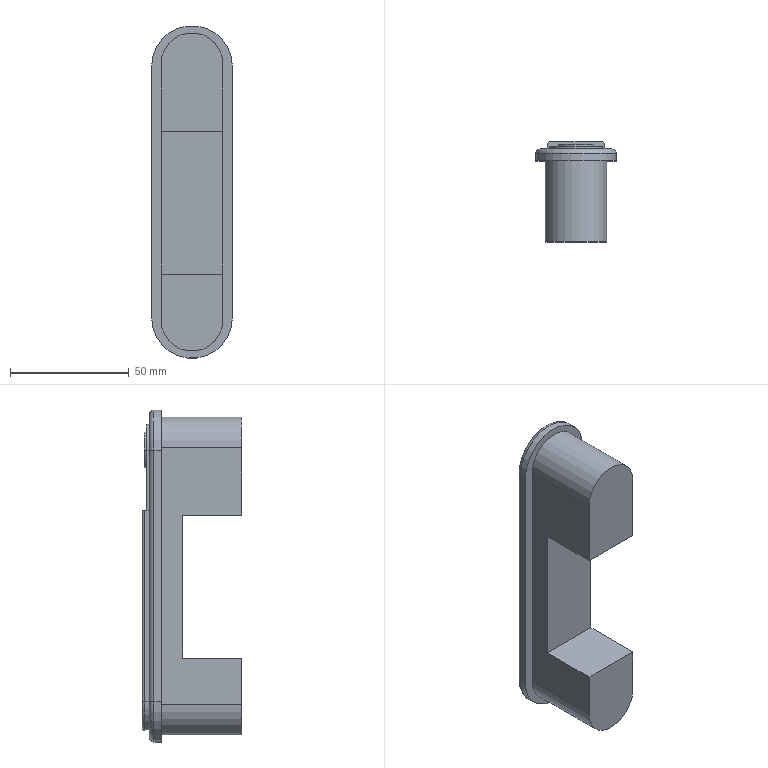Component | SolidWorks | OuterDoorAssembly1-1_MMS480-2A-1Lock-1 | 1 solid | 39 faces | box 34 x 42.01 x 140 mm | volume 104134 mm3 | plane 24 | cylinder 12 | torus 3 | commonest cylinder face diameters 15 x2 34 x2 4 x2 2 x2 26 x2 24 x1 22 x1
STEP:
#1=CARTESIAN_POINT('',(-2.264,7.503,34.753));
#2=VERTEX_POINT('',#1);
#3=CARTESIAN_POINT('',(-2.854,7.503,34.753));
#4=VERTEX_POINT('',#3);
#5=CARTESIAN_POINT('',(-2.559,7.503,34.753));
#6=DIRECTION('',(0.0003491,1.,-0.));
#7=DIRECTION('',(1.,-0.0003491,0.));
#8=AXIS2_PLACEMENT_3D('',#5,#6,#7);
#9=CIRCLE('',#8,0.2953);
#10=EDGE_CURVE('',#2,#4,#9,.T.);
#11=ORIENTED_EDGE('',*,*,#10,.F.);
#12=CARTESIAN_POINT('',(-2.264,7.463,34.753));
#13=VERTEX_POINT('',#12);
#14=CARTESIAN_POINT('',(-2.264,7.503,34.753));
#15=DIRECTION('',(-0.0003491,-1.,0.));
#16=VECTOR('',#15,39.37);
#17=LINE('',#14,#16);
#18=EDGE_CURVE('',#2,#13,#17,.T.);
#19=ORIENTED_EDGE('',*,*,#18,.T.);
#20=CARTESIAN_POINT('',(-2.854,7.463,34.753));
#21=VERTEX_POINT('',#20);
#22=CARTESIAN_POINT('',(-2.559,7.463,34.753));
#23=DIRECTION('',(0.0003491,1.,-0.));
#24=DIRECTION('',(1.,-0.0003491,0.));
#25=AXIS2_PLACEMENT_3D('',#22,#23,#24);
#26=CIRCLE('',#25,0.2953);
#27=EDGE_CURVE('',#13,#21,#26,.T.);
#28=ORIENTED_EDGE('',*,*,#27,.T.);
#29=CARTESIAN_POINT('',(-2.854,7.503,34.753));
#30=DIRECTION('',(-0.0003491,-1.,0.));
#31=VECTOR('',#30,39.37);
#32=LINE('',#29,#31);
#33=EDGE_CURVE('',#4,#21,#32,.T.);
#34=ORIENTED_EDGE('',*,*,#33,.F.);
#35=EDGE_LOOP('',(#11,#19,#28,#34));
#36=FACE_OUTER_BOUND('',#35,.T.);
#37=CARTESIAN_POINT('',(-2.559,7.503,34.753));
#38=DIRECTION('',(-0.0003491,-1.,0.));
#39=DIRECTION('',(-1.,0.0003491,0.));
#40=AXIS2_PLACEMENT_3D('',#37,#38,#39);
#41=CYLINDRICAL_SURFACE('',#40,0.2953);
#42=ADVANCED_FACE('',(#36),#41,.T.);
#43=CARTESIAN_POINT('',(-2.048,5.888,30.54));
#44=VERTEX_POINT('',#43);
#45=CARTESIAN_POINT('',(-2.048,5.888,31.307));
#46=VERTEX_POINT('',#45);
#47=CARTESIAN_POINT('',(-2.048,5.888,30.54));
#48=DIRECTION('',(-0.,0.,1.));
#49=VECTOR('',#48,39.37);
#50=LINE('',#47,#49);
#51=EDGE_CURVE('',#44,#46,#50,.T.);
#52=ORIENTED_EDGE('',*,*,#51,.T.);
#53=CARTESIAN_POINT('',(-3.071,5.889,31.307));
#54=VERTEX_POINT('',#53);
#55=CARTESIAN_POINT('',(-2.56,5.888,31.307));
#56=DIRECTION('',(1.,-0.0003491,0.));
#57=VECTOR('',#56,39.37);
#58=LINE('',#55,#57);
#59=EDGE_CURVE('',#54,#46,#58,.T.);
#60=ORIENTED_EDGE('',*,*,#59,.F.);
#61=CARTESIAN_POINT('',(-3.071,5.889,30.54));
#62=VERTEX_POINT('',#61);
#63=CARTESIAN_POINT('',(-3.071,5.889,30.54));
#64=DIRECTION('',(0.,-0.,-1.));
#65=VECTOR('',#64,39.37);
#66=LINE('',#63,#65);
#67=EDGE_CURVE('',#54,#62,#66,.T.);
#68=ORIENTED_EDGE('',*,*,#67,.T.);
#69=CARTESIAN_POINT('',(-2.56,5.888,30.54));
#70=DIRECTION('',(-0.0003491,-1.,0.));
#71=DIRECTION('',(-1.,0.0003491,0.));
#72=AXIS2_PLACEMENT_3D('',#69,#70,#71);
#73=CIRCLE('',#72,0.5118);
#74=EDGE_CURVE('',#62,#44,#73,.T.);
#75=ORIENTED_EDGE('',*,*,#74,.T.);
#76=EDGE_LOOP('',(#52,#60,#68,#75));
#77=FACE_OUTER_BOUND('',#76,.T.);
#78=CARTESIAN_POINT('',(-2.56,5.888,30.54));
#79=DIRECTION('',(-0.0003491,-1.,0.));
#80=DIRECTION('',(-1.,0.0003491,-0.));
#81=AXIS2_PLACEMENT_3D('',#78,#79,#80);
#82=PLANE('',#81);
#83=ADVANCED_FACE('',(#77),#82,.T.);
#84=CARTESIAN_POINT('',(-1.89,7.227,30.58));
#85=VERTEX_POINT('',#84);
#86=CARTESIAN_POINT('',(-3.228,7.227,30.58));
#87=VERTEX_POINT('',#86);
#88=CARTESIAN_POINT('',(-2.559,7.227,30.58));
#89=DIRECTION('',(0.0003491,1.,-0.));
#90=DIRECTION('',(1.,-0.0003491,0.));
#91=AXIS2_PLACEMENT_3D('',#88,#89,#90);
#92=CIRCLE('',#91,0.6693);
#93=EDGE_CURVE('',#85,#87,#92,.T.);
#94=ORIENTED_EDGE('',*,*,#93,.F.);
#95=CARTESIAN_POINT('',(-1.89,7.227,34.753));
#96=VERTEX_POINT('',#95);
#97=CARTESIAN_POINT('',(-1.89,7.227,30.58));
#98=DIRECTION('',(0.,-0.,-1.));
#99=VECTOR('',#98,39.37);
#100=LINE('',#97,#99);
#101=EDGE_CURVE('',#96,#85,#100,.T.);
#102=ORIENTED_EDGE('',*,*,#101,.F.);
#103=CARTESIAN_POINT('',(-3.228,7.227,34.753));
#104=VERTEX_POINT('',#103);
#105=CARTESIAN_POINT('',(-2.559,7.227,34.753));
#106=DIRECTION('',(0.0003491,1.,-0.));
#107=DIRECTION('',(1.,-0.0003491,0.));
#108=AXIS2_PLACEMENT_3D('',#105,#106,#107);
#109=CIRCLE('',#108,0.6693);
#110=EDGE_CURVE('',#104,#96,#109,.T.);
#111=ORIENTED_EDGE('',*,*,#110,.F.);
#112=CARTESIAN_POINT('',(-3.228,7.227,30.58));
#113=DIRECTION('',(-0.,0.,1.));
#114=VECTOR('',#113,39.37);
#115=LINE('',#112,#114);
#116=EDGE_CURVE('',#87,#104,#115,.T.);
#117=ORIENTED_EDGE('',*,*,#116,.F.);
#118=EDGE_LOOP('',(#94,#102,#111,#117));
#119=FACE_OUTER_BOUND('',#118,.T.);
#120=CARTESIAN_POINT('',(-3.071,7.227,30.54));
#121=VERTEX_POINT('',#120);
#122=CARTESIAN_POINT('',(-2.047,7.227,30.54));
#123=VERTEX_POINT('',#122);
#124=CARTESIAN_POINT('',(-2.559,7.227,30.54));
#125=DIRECTION('',(-0.0003491,-1.,0.));
#126=DIRECTION('',(-1.,0.0003491,0.));
#127=AXIS2_PLACEMENT_3D('',#124,#125,#126);
#128=CIRCLE('',#127,0.5118);
#129=EDGE_CURVE('',#121,#123,#128,.T.);
#130=ORIENTED_EDGE('',*,*,#129,.F.);
#131=CARTESIAN_POINT('',(-3.071,7.227,34.792));
#132=VERTEX_POINT('',#131);
#133=CARTESIAN_POINT('',(-3.071,7.227,30.54));
#134=DIRECTION('',(0.,-0.,-1.));
#135=VECTOR('',#134,39.37);
#136=LINE('',#133,#135);
#137=EDGE_CURVE('',#132,#121,#136,.T.);
#138=ORIENTED_EDGE('',*,*,#137,.F.);
#139=CARTESIAN_POINT('',(-2.047,7.227,34.792));
#140=VERTEX_POINT('',#139);
#141=CARTESIAN_POINT('',(-2.559,7.227,34.792));
#142=DIRECTION('',(-0.0003491,-1.,0.));
#143=DIRECTION('',(-1.,0.0003491,0.));
#144=AXIS2_PLACEMENT_3D('',#141,#142,#143);
#145=CIRCLE('',#144,0.5118);
#146=EDGE_CURVE('',#140,#132,#145,.T.);
#147=ORIENTED_EDGE('',*,*,#146,.F.);
#148=CARTESIAN_POINT('',(-2.047,7.227,30.54));
#149=DIRECTION('',(-0.,0.,1.));
#150=VECTOR('',#149,39.37);
#151=LINE('',#148,#150);
#152=EDGE_CURVE('',#123,#140,#151,.T.);
#153=ORIENTED_EDGE('',*,*,#152,.F.);
#154=EDGE_LOOP('',(#130,#138,#147,#153));
#155=FACE_BOUND('',#154,.T.);
#156=CARTESIAN_POINT('',(-2.559,7.227,30.58));
#157=DIRECTION('',(0.0003491,1.,-0.));
#158=DIRECTION('',(1.,-0.0003491,0.));
#159=AXIS2_PLACEMENT_3D('',#156,#157,#158);
#160=PLANE('',#159);
#161=ADVANCED_FACE('',(#119,#155),#160,.F.);
#162=CARTESIAN_POINT('',(-2.992,7.463,33.745));
#163=VERTEX_POINT('',#162);
#164=CARTESIAN_POINT('',(-2.126,7.463,33.745));
#165=VERTEX_POINT('',#164);
#166=CARTESIAN_POINT('',(-3.031,7.463,33.745));
#167=DIRECTION('',(1.,-0.0003491,0.));
#168=VECTOR('',#167,39.37);
#169=LINE('',#166,#168);
#170=EDGE_CURVE('',#163,#165,#169,.T.);
#171=ORIENTED_EDGE('',*,*,#170,.F.);
#172=CARTESIAN_POINT('',(-2.992,7.463,34.753));
#173=VERTEX_POINT('',#172);
#174=CARTESIAN_POINT('',(-2.992,7.463,34.753));
#175=DIRECTION('',(-0.,0.,1.));
#176=VECTOR('',#175,39.37);
#177=LINE('',#174,#176);
#178=EDGE_CURVE('',#163,#173,#177,.T.);
#179=ORIENTED_EDGE('',*,*,#178,.T.);
#180=CARTESIAN_POINT('',(-2.126,7.463,34.753));
#181=VERTEX_POINT('',#180);
#182=CARTESIAN_POINT('',(-2.559,7.463,34.753));
#183=DIRECTION('',(0.0003491,1.,-0.));
#184=DIRECTION('',(1.,-0.0003491,0.));
#185=AXIS2_PLACEMENT_3D('',#182,#183,#184);
#186=CIRCLE('',#185,0.4331);
#187=EDGE_CURVE('',#173,#181,#186,.T.);
#188=ORIENTED_EDGE('',*,*,#187,.T.);
#189=CARTESIAN_POINT('',(-2.126,7.463,34.753));
#190=DIRECTION('',(0.,-0.,-1.));
#191=VECTOR('',#190,39.37);
#192=LINE('',#189,#191);
#193=EDGE_CURVE('',#181,#165,#192,.T.);
#194=ORIENTED_EDGE('',*,*,#193,.T.);
#195=EDGE_LOOP('',(#171,#179,#188,#194));
#196=FACE_OUTER_BOUND('',#195,.T.);
#197=CARTESIAN_POINT('',(-2.559,7.463,34.753));
#198=DIRECTION('',(0.0003491,1.,-0.));
#199=DIRECTION('',(1.,-0.0003491,0.));
#200=AXIS2_PLACEMENT_3D('',#197,#198,#199);
#201=CIRCLE('',#200,0.2953);
#202=EDGE_CURVE('',#21,#13,#201,.T.);
#203=ORIENTED_EDGE('',*,*,#202,.F.);
#204=ORIENTED_EDGE('',*,*,#27,.F.);
#205=EDGE_LOOP('',(#203,#204));
#206=FACE_BOUND('',#205,.T.);
#207=CARTESIAN_POINT('',(-2.559,7.463,34.753));
#208=DIRECTION('',(0.0003491,1.,-0.));
#209=DIRECTION('',(1.,-0.0003491,0.));
#210=AXIS2_PLACEMENT_3D('',#207,#208,#209);
#211=PLANE('',#210);
#212=ADVANCED_FACE('',(#196,#206),#211,.T.);
#213=CARTESIAN_POINT('',(-3.15,7.424,34.753));
#214=VERTEX_POINT('',#213);
#215=CARTESIAN_POINT('',(-1.968,7.424,34.753));
#216=VERTEX_POINT('',#215);
#217=CARTESIAN_POINT('',(-2.559,7.424,34.753));
#218=DIRECTION('',(0.0003491,1.,-0.));
#219=DIRECTION('',(1.,-0.0003491,0.));
#220=AXIS2_PLACEMENT_3D('',#217,#218,#219);
#221=CIRCLE('',#220,0.5906);
#222=EDGE_CURVE('',#214,#216,#221,.T.);
#223=ORIENTED_EDGE('',*,*,#222,.T.);
#224=CARTESIAN_POINT('',(-1.968,7.424,30.58));
#225=VERTEX_POINT('',#224);
#226=CARTESIAN_POINT('',(-1.968,7.424,30.58));
#227=DIRECTION('',(0.,-0.,-1.));
#228=VECTOR('',#227,39.37);
#229=LINE('',#226,#228);
#230=EDGE_CURVE('',#216,#225,#229,.T.);
#231=ORIENTED_EDGE('',*,*,#230,.T.);
#232=CARTESIAN_POINT('',(-3.15,7.424,30.58));
#233=VERTEX_POINT('',#232);
#234=CARTESIAN_POINT('',(-2.559,7.424,30.58));
#235=DIRECTION('',(0.0003491,1.,-0.));
#236=DIRECTION('',(1.,-0.0003491,0.));
#237=AXIS2_PLACEMENT_3D('',#234,#235,#236);
#238=CIRCLE('',#237,0.5906);
#239=EDGE_CURVE('',#225,#233,#238,.T.);
#240=ORIENTED_EDGE('',*,*,#239,.T.);
#241=CARTESIAN_POINT('',(-3.15,7.424,34.753));
#242=DIRECTION('',(-0.,0.,1.));
#243=VECTOR('',#242,39.37);
#244=LINE('',#241,#243);
#245=EDGE_CURVE('',#233,#214,#244,.T.);
#246=ORIENTED_EDGE('',*,*,#245,.T.);
#247=EDGE_LOOP('',(#223,#231,#240,#246));
#248=FACE_OUTER_BOUND('',#247,.T.);
#249=CARTESIAN_POINT('',(-2.126,7.424,33.745));
#250=VERTEX_POINT('',#249);
#251=CARTESIAN_POINT('',(-2.087,7.424,33.745));
#252=VERTEX_POINT('',#251);
#253=CARTESIAN_POINT('',(-3.031,7.424,33.745));
#254=DIRECTION('',(1.,-0.0003491,0.));
#255=VECTOR('',#254,39.37);
#256=LINE('',#253,#255);
#257=EDGE_CURVE('',#250,#252,#256,.T.);
#258=ORIENTED_EDGE('',*,*,#257,.F.);
#259=CARTESIAN_POINT('',(-2.126,7.424,34.753));
#260=VERTEX_POINT('',#259);
#261=CARTESIAN_POINT('',(-2.126,7.424,34.753));
#262=DIRECTION('',(0.,-0.,-1.));
#263=VECTOR('',#262,39.37);
#264=LINE('',#261,#263);
#265=EDGE_CURVE('',#260,#250,#264,.T.);
#266=ORIENTED_EDGE('',*,*,#265,.F.);
#267=CARTESIAN_POINT('',(-2.992,7.424,34.753));
#268=VERTEX_POINT('',#267);
#269=CARTESIAN_POINT('',(-2.559,7.424,34.753));
#270=DIRECTION('',(0.0003491,1.,-0.));
#271=DIRECTION('',(1.,-0.0003491,0.));
#272=AXIS2_PLACEMENT_3D('',#269,#270,#271);
#273=CIRCLE('',#272,0.4331);
#274=EDGE_CURVE('',#268,#260,#273,.T.);
#275=ORIENTED_EDGE('',*,*,#274,.F.);
#276=CARTESIAN_POINT('',(-2.992,7.424,33.745));
#277=VERTEX_POINT('',#276);
#278=CARTESIAN_POINT('',(-2.992,7.424,34.753));
#279=DIRECTION('',(-0.,0.,1.));
#280=VECTOR('',#279,39.37);
#281=LINE('',#278,#280);
#282=EDGE_CURVE('',#277,#268,#281,.T.);
#283=ORIENTED_EDGE('',*,*,#282,.F.);
#284=CARTESIAN_POINT('',(-3.031,7.424,33.745));
#285=VERTEX_POINT('',#284);
#286=CARTESIAN_POINT('',(-3.031,7.424,33.745));
#287=DIRECTION('',(1.,-0.0003491,0.));
#288=VECTOR('',#287,39.37);
#289=LINE('',#286,#288);
#290=EDGE_CURVE('',#285,#277,#289,.T.);
#291=ORIENTED_EDGE('',*,*,#290,.F.);
#292=CARTESIAN_POINT('',(-3.031,7.424,30.58));
#293=VERTEX_POINT('',#292);
#294=CARTESIAN_POINT('',(-3.031,7.424,30.58));
#295=DIRECTION('',(-0.,0.,1.));
#296=VECTOR('',#295,39.37);
#297=LINE('',#294,#296);
#298=EDGE_CURVE('',#293,#285,#297,.T.);
#299=ORIENTED_EDGE('',*,*,#298,.F.);
#300=CARTESIAN_POINT('',(-2.087,7.424,30.58));
#301=VERTEX_POINT('',#300);
#302=CARTESIAN_POINT('',(-2.559,7.424,30.58));
#303=DIRECTION('',(0.0003491,1.,-0.));
#304=DIRECTION('',(1.,-0.0003491,0.));
#305=AXIS2_PLACEMENT_3D('',#302,#303,#304);
#306=CIRCLE('',#305,0.4724);
#307=EDGE_CURVE('',#301,#293,#306,.T.);
#308=ORIENTED_EDGE('',*,*,#307,.F.);
#309=CARTESIAN_POINT('',(-2.087,7.424,30.58));
#310=DIRECTION('',(0.,-0.,-1.));
#311=VECTOR('',#310,39.37);
#312=LINE('',#309,#311);
#313=EDGE_CURVE('',#252,#301,#312,.T.);
#314=ORIENTED_EDGE('',*,*,#313,.F.);
#315=EDGE_LOOP('',(#258,#266,#275,#283,#291,#299,#308,#314));
#316=FACE_BOUND('',#315,.T.);
#317=CARTESIAN_POINT('',(-2.559,7.424,30.58));
#318=DIRECTION('',(0.0003491,1.,-0.));
#319=DIRECTION('',(1.,-0.0003491,0.));
#320=AXIS2_PLACEMENT_3D('',#317,#318,#319);
#321=PLANE('',#320);
#322=ADVANCED_FACE('',(#248,#316),#321,.T.);
#323=CARTESIAN_POINT('',(-2.087,7.502,33.745));
#324=VERTEX_POINT('',#323);
#325=CARTESIAN_POINT('',(-2.087,7.542,33.745));
#326=DIRECTION('',(-0.0003491,-1.,0.));
#327=VECTOR('',#326,39.37);
#328=LINE('',#325,#327);
#329=EDGE_CURVE('',#324,#252,#328,.T.);
#330=ORIENTED_EDGE('',*,*,#329,.F.);
#331=CARTESIAN_POINT('',(-2.126,7.542,33.745));
#332=VERTEX_POINT('',#331);
#333=CARTESIAN_POINT('',(-2.126,7.502,33.745));
#334=DIRECTION('',(-0.,0.,1.));
#335=DIRECTION('',(0.0003491,1.,0.));
#336=AXIS2_PLACEMENT_3D('',#333,#334,#335);
#337=CIRCLE('',#336,0.03937);
#338=EDGE_CURVE('',#324,#332,#337,.T.);
#339=ORIENTED_EDGE('',*,*,#338,.T.);
#340=CARTESIAN_POINT('',(-2.992,7.542,33.745));
#341=VERTEX_POINT('',#340);
#342=CARTESIAN_POINT('',(-3.031,7.542,33.745));
#343=DIRECTION('',(1.,-0.0003491,0.));
#344=VECTOR('',#343,39.37);
#345=LINE('',#342,#344);
#346=EDGE_CURVE('',#341,#332,#345,.T.);
#347=ORIENTED_EDGE('',*,*,#346,.F.);
#348=CARTESIAN_POINT('',(-3.031,7.503,33.745));
#349=VERTEX_POINT('',#348);
#350=CARTESIAN_POINT('',(-2.992,7.503,33.745));
#351=DIRECTION('',(-0.,0.,1.));
#352=DIRECTION('',(0.0003491,1.,0.));
#353=AXIS2_PLACEMENT_3D('',#350,#351,#352);
#354=CIRCLE('',#353,0.03937);
#355=EDGE_CURVE('',#341,#349,#354,.T.);
#356=ORIENTED_EDGE('',*,*,#355,.T.);
#357=CARTESIAN_POINT('',(-3.031,7.542,33.745));
#358=DIRECTION('',(-0.0003491,-1.,0.));
#359=VECTOR('',#358,39.37);
#360=LINE('',#357,#359);
#361=EDGE_CURVE('',#349,#285,#360,.T.);
#362=ORIENTED_EDGE('',*,*,#361,.T.);
#363=ORIENTED_EDGE('',*,*,#290,.T.);
#364=CARTESIAN_POINT('',(-2.992,7.542,33.745));
#365=DIRECTION('',(-0.0003491,-1.,0.));
#366=VECTOR('',#365,39.37);
#367=LINE('',#364,#366);
#368=EDGE_CURVE('',#163,#277,#367,.T.);
#369=ORIENTED_EDGE('',*,*,#368,.F.);
#370=ORIENTED_EDGE('',*,*,#170,.T.);
#371=CARTESIAN_POINT('',(-2.126,7.542,33.745));
#372=DIRECTION('',(0.0003491,1.,-0.));
#373=VECTOR('',#372,39.37);
#374=LINE('',#371,#373);
#375=EDGE_CURVE('',#250,#165,#374,.T.);
#376=ORIENTED_EDGE('',*,*,#375,.F.);
#377=ORIENTED_EDGE('',*,*,#257,.T.);
#378=EDGE_LOOP('',(#330,#339,#347,#356,#362,#363,#369,#370,#376,#377));
#379=FACE_OUTER_BOUND('',#378,.T.);
#380=CARTESIAN_POINT('',(-3.031,7.542,33.745));
#381=DIRECTION('',(0.,-0.,-1.));
#382=DIRECTION('',(0.0003491,1.,-0.));
#383=AXIS2_PLACEMENT_3D('',#380,#381,#382);
#384=PLANE('',#383);
#385=ADVANCED_FACE('',(#379),#384,.F.);
#386=CARTESIAN_POINT('',(-3.228,7.345,30.58));
#387=VERTEX_POINT('',#386);
#388=CARTESIAN_POINT('',(-3.228,7.424,30.58));
#389=DIRECTION('',(-0.0003491,-1.,0.));
#390=VECTOR('',#389,39.37);
#391=LINE('',#388,#390);
#392=EDGE_CURVE('',#387,#87,#391,.T.);
#393=ORIENTED_EDGE('',*,*,#392,.F.);
#394=CARTESIAN_POINT('',(-1.89,7.345,30.58));
#395=VERTEX_POINT('',#394);
#396=CARTESIAN_POINT('',(-2.559,7.345,30.58));
#397=DIRECTION('',(-0.0003491,-1.,0.));
#398=DIRECTION('',(1.,-0.0003491,0.));
#399=AXIS2_PLACEMENT_3D('',#396,#397,#398);
#400=CIRCLE('',#399,0.6693);
#401=EDGE_CURVE('',#387,#395,#400,.T.);
#402=ORIENTED_EDGE('',*,*,#401,.T.);
#403=CARTESIAN_POINT('',(-1.89,7.424,30.58));
#404=DIRECTION('',(-0.0003491,-1.,0.));
#405=VECTOR('',#404,39.37);
#406=LINE('',#403,#405);
#407=EDGE_CURVE('',#395,#85,#406,.T.);
#408=ORIENTED_EDGE('',*,*,#407,.T.);
#409=ORIENTED_EDGE('',*,*,#93,.T.);
#410=EDGE_LOOP('',(#393,#402,#408,#409));
#411=FACE_OUTER_BOUND('',#410,.T.);
#412=CARTESIAN_POINT('',(-2.559,7.424,30.58));
#413=DIRECTION('',(-0.0003491,-1.,0.));
#414=DIRECTION('',(-1.,0.0003491,-0.));
#415=AXIS2_PLACEMENT_3D('',#412,#413,#414);
#416=CYLINDRICAL_SURFACE('',#415,0.6693);
#417=ADVANCED_FACE('',(#411),#416,.T.);
#418=CARTESIAN_POINT('',(-3.228,7.345,34.753));
#419=VERTEX_POINT('',#418);
#420=CARTESIAN_POINT('',(-3.228,7.424,34.753));
#421=DIRECTION('',(-0.0003491,-1.,0.));
#422=VECTOR('',#421,39.37);
#423=LINE('',#420,#422);
#424=EDGE_CURVE('',#419,#104,#423,.T.);
#425=ORIENTED_EDGE('',*,*,#424,.F.);
#426=CARTESIAN_POINT('',(-3.228,7.345,30.58));
#427=DIRECTION('',(0.,-0.,-1.));
#428=VECTOR('',#427,39.37);
#429=LINE('',#426,#428);
#430=EDGE_CURVE('',#419,#387,#429,.T.);
#431=ORIENTED_EDGE('',*,*,#430,.T.);
#432=ORIENTED_EDGE('',*,*,#392,.T.);
#433=ORIENTED_EDGE('',*,*,#116,.T.);
#434=EDGE_LOOP('',(#425,#431,#432,#433));
#435=FACE_OUTER_BOUND('',#434,.T.);
#436=CARTESIAN_POINT('',(-3.228,7.424,30.58));
#437=DIRECTION('',(1.,-0.0003491,0.));
#438=DIRECTION('',(0.,-0.,-1.));
#439=AXIS2_PLACEMENT_3D('',#436,#437,#438);
#440=PLANE('',#439);
#441=ADVANCED_FACE('',(#435),#440,.F.);
#442=CARTESIAN_POINT('',(-1.89,7.345,34.753));
#443=VERTEX_POINT('',#442);
#444=CARTESIAN_POINT('',(-1.89,7.424,34.753));
#445=DIRECTION('',(-0.0003491,-1.,0.));
#446=VECTOR('',#445,39.37);
#447=LINE('',#444,#446);
#448=EDGE_CURVE('',#443,#96,#447,.T.);
#449=ORIENTED_EDGE('',*,*,#448,.F.);
#450=CARTESIAN_POINT('',(-2.559,7.345,34.753));
#451=DIRECTION('',(-0.0003491,-1.,0.));
#452=DIRECTION('',(1.,-0.0003491,0.));
#453=AXIS2_PLACEMENT_3D('',#450,#451,#452);
#454=CIRCLE('',#453,0.6693);
#455=EDGE_CURVE('',#443,#419,#454,.T.);
#456=ORIENTED_EDGE('',*,*,#455,.T.);
#457=ORIENTED_EDGE('',*,*,#424,.T.);
#458=ORIENTED_EDGE('',*,*,#110,.T.);
#459=EDGE_LOOP('',(#449,#456,#457,#458));
#460=FACE_OUTER_BOUND('',#459,.T.);
#461=CARTESIAN_POINT('',(-2.559,7.424,34.753));
#462=DIRECTION('',(-0.0003491,-1.,0.));
#463=DIRECTION('',(-1.,0.0003491,-0.));
#464=AXIS2_PLACEMENT_3D('',#461,#462,#463);
#465=CYLINDRICAL_SURFACE('',#464,0.6693);
#466=ADVANCED_FACE('',(#460),#465,.T.);
#467=ORIENTED_EDGE('',*,*,#407,.F.);
#468=CARTESIAN_POINT('',(-1.89,7.345,34.753));
#469=DIRECTION('',(-0.,0.,1.));
#470=VECTOR('',#469,39.37);
#471=LINE('',#468,#470);
#472=EDGE_CURVE('',#395,#443,#471,.T.);
#473=ORIENTED_EDGE('',*,*,#472,.T.);
#474=ORIENTED_EDGE('',*,*,#448,.T.);
#475=ORIENTED_EDGE('',*,*,#101,.T.);
#476=EDGE_LOOP('',(#467,#473,#474,#475));
#477=FACE_OUTER_BOUND('',#476,.T.);
#478=CARTESIAN_POINT('',(-1.89,7.424,30.58));
#479=DIRECTION('',(-1.,0.0003491,-0.));
#480=DIRECTION('',(-0.,0.,1.));
#481=AXIS2_PLACEMENT_3D('',#478,#479,#480);
#482=PLANE('',#481);
#483=ADVANCED_FACE('',(#477),#482,.F.);
#484=CARTESIAN_POINT('',(-3.031,7.503,30.58));
#485=VERTEX_POINT('',#484);
#486=CARTESIAN_POINT('',(-3.031,7.542,30.58));
#487=DIRECTION('',(-0.0003491,-1.,0.));
#488=VECTOR('',#487,39.37);
#489=LINE('',#486,#488);
#490=EDGE_CURVE('',#485,#293,#489,.T.);
#491=ORIENTED_EDGE('',*,*,#490,.F.);
#492=CARTESIAN_POINT('',(-2.087,7.502,30.58));
#493=VERTEX_POINT('',#492);
#494=CARTESIAN_POINT('',(-2.559,7.503,30.58));
#495=DIRECTION('',(-0.0003491,-1.,0.));
#496=DIRECTION('',(1.,-0.0003491,0.));
#497=AXIS2_PLACEMENT_3D('',#494,#495,#496);
#498=CIRCLE('',#497,0.4724);
#499=EDGE_CURVE('',#485,#493,#498,.T.);
#500=ORIENTED_EDGE('',*,*,#499,.T.);
#501=CARTESIAN_POINT('',(-2.087,7.542,30.58));
#502=DIRECTION('',(-0.0003491,-1.,0.));
#503=VECTOR('',#502,39.37);
#504=LINE('',#501,#503);
#505=EDGE_CURVE('',#493,#301,#504,.T.);
#506=ORIENTED_EDGE('',*,*,#505,.T.);
#507=ORIENTED_EDGE('',*,*,#307,.T.);
#508=EDGE_LOOP('',(#491,#500,#506,#507));
#509=FACE_OUTER_BOUND('',#508,.T.);
#510=CARTESIAN_POINT('',(-2.559,7.542,30.58));
#511=DIRECTION('',(-0.0003491,-1.,0.));
#512=DIRECTION('',(-1.,0.0003491,0.));
#513=AXIS2_PLACEMENT_3D('',#510,#511,#512);
#514=CYLINDRICAL_SURFACE('',#513,0.4724);
#515=ADVANCED_FACE('',(#509),#514,.T.);
#516=ORIENTED_EDGE('',*,*,#361,.F.);
#517=CARTESIAN_POINT('',(-3.031,7.503,30.58));
#518=DIRECTION('',(0.,-0.,-1.));
#519=VECTOR('',#518,39.37);
#520=LINE('',#517,#519);
#521=EDGE_CURVE('',#349,#485,#520,.T.);
#522=ORIENTED_EDGE('',*,*,#521,.T.);
#523=ORIENTED_EDGE('',*,*,#490,.T.);
#524=ORIENTED_EDGE('',*,*,#298,.T.);
#525=EDGE_LOOP('',(#516,#522,#523,#524));
#526=FACE_OUTER_BOUND('',#525,.T.);
#527=CARTESIAN_POINT('',(-3.031,7.542,30.58));
#528=DIRECTION('',(1.,-0.0003491,0.));
#529=DIRECTION('',(-0.0003491,-1.,0.));
#530=AXIS2_PLACEMENT_3D('',#527,#528,#529);
#531=PLANE('',#530);
#532=ADVANCED_FACE('',(#526),#531,.F.);
#533=ORIENTED_EDGE('',*,*,#505,.F.);
#534=CARTESIAN_POINT('',(-2.087,7.502,33.745));
#535=DIRECTION('',(-0.,0.,1.));
#536=VECTOR('',#535,39.37);
#537=LINE('',#534,#536);
#538=EDGE_CURVE('',#493,#324,#537,.T.);
#539=ORIENTED_EDGE('',*,*,#538,.T.);
#540=ORIENTED_EDGE('',*,*,#329,.T.);
#541=ORIENTED_EDGE('',*,*,#313,.T.);
#542=EDGE_LOOP('',(#533,#539,#540,#541));
#543=FACE_OUTER_BOUND('',#542,.T.);
#544=CARTESIAN_POINT('',(-2.087,7.542,30.58));
#545=DIRECTION('',(-1.,0.0003491,-0.));
#546=DIRECTION('',(0.0003491,1.,-0.));
#547=AXIS2_PLACEMENT_3D('',#544,#545,#546);
#548=PLANE('',#547);
#549=ADVANCED_FACE('',(#543),#548,.F.);
#550=ORIENTED_EDGE('',*,*,#346,.T.);
#551=CARTESIAN_POINT('',(-2.126,7.542,30.58));
#552=VERTEX_POINT('',#551);
#553=CARTESIAN_POINT('',(-2.126,7.542,30.58));
#554=DIRECTION('',(0.,-0.,-1.));
#555=VECTOR('',#554,39.37);
#556=LINE('',#553,#555);
#557=EDGE_CURVE('',#332,#552,#556,.T.);
#558=ORIENTED_EDGE('',*,*,#557,.T.);
#559=CARTESIAN_POINT('',(-2.992,7.542,30.58));
#560=VERTEX_POINT('',#559);
#561=CARTESIAN_POINT('',(-2.559,7.542,30.58));
#562=DIRECTION('',(0.0003491,1.,-0.));
#563=DIRECTION('',(1.,-0.0003491,0.));
#564=AXIS2_PLACEMENT_3D('',#561,#562,#563);
#565=CIRCLE('',#564,0.4331);
#566=EDGE_CURVE('',#552,#560,#565,.T.);
#567=ORIENTED_EDGE('',*,*,#566,.T.);
#568=CARTESIAN_POINT('',(-2.992,7.542,33.745));
#569=DIRECTION('',(-0.,0.,1.));
#570=VECTOR('',#569,39.37);
#571=LINE('',#568,#570);
#572=EDGE_CURVE('',#560,#341,#571,.T.);
#573=ORIENTED_EDGE('',*,*,#572,.T.);
#574=EDGE_LOOP('',(#550,#558,#567,#573));
#575=FACE_OUTER_BOUND('',#574,.T.);
#576=CARTESIAN_POINT('',(-2.559,7.542,30.58));
#577=DIRECTION('',(0.0003491,1.,-0.));
#578=DIRECTION('',(1.,-0.0003491,0.));
#579=AXIS2_PLACEMENT_3D('',#576,#577,#578);
#580=PLANE('',#579);
#581=ADVANCED_FACE('',(#575),#580,.T.);
#582=ORIENTED_EDGE('',*,*,#265,.T.);
#583=ORIENTED_EDGE('',*,*,#375,.T.);
#584=ORIENTED_EDGE('',*,*,#193,.F.);
#585=CARTESIAN_POINT('',(-2.126,7.463,34.753));
#586=DIRECTION('',(-0.0003491,-1.,0.));
#587=VECTOR('',#586,39.37);
#588=LINE('',#585,#587);
#589=EDGE_CURVE('',#181,#260,#588,.T.);
#590=ORIENTED_EDGE('',*,*,#589,.T.);
#591=EDGE_LOOP('',(#582,#583,#584,#590));
#592=FACE_OUTER_BOUND('',#591,.T.);
#593=CARTESIAN_POINT('',(-2.126,7.463,34.753));
#594=DIRECTION('',(-1.,0.0003491,-0.));
#595=DIRECTION('',(0.0003491,1.,-0.));
#596=AXIS2_PLACEMENT_3D('',#593,#594,#595);
#597=PLANE('',#596);
#598=ADVANCED_FACE('',(#592),#597,.F.);
#599=ORIENTED_EDGE('',*,*,#178,.F.);
#600=ORIENTED_EDGE('',*,*,#368,.T.);
#601=ORIENTED_EDGE('',*,*,#282,.T.);
#602=CARTESIAN_POINT('',(-2.992,7.463,34.753));
#603=DIRECTION('',(-0.0003491,-1.,0.));
#604=VECTOR('',#603,39.37);
#605=LINE('',#602,#604);
#606=EDGE_CURVE('',#173,#268,#605,.T.);
#607=ORIENTED_EDGE('',*,*,#606,.F.);
#608=EDGE_LOOP('',(#599,#600,#601,#607));
#609=FACE_OUTER_BOUND('',#608,.T.);
#610=CARTESIAN_POINT('',(-2.992,7.463,34.753));
#611=DIRECTION('',(1.,-0.0003491,0.));
#612=DIRECTION('',(-0.0003491,-1.,0.));
#613=AXIS2_PLACEMENT_3D('',#610,#611,#612);
#614=PLANE('',#613);
#615=ADVANCED_FACE('',(#609),#614,.F.);
#616=ORIENTED_EDGE('',*,*,#274,.T.);
#617=ORIENTED_EDGE('',*,*,#589,.F.);
#618=ORIENTED_EDGE('',*,*,#187,.F.);
#619=ORIENTED_EDGE('',*,*,#606,.T.);
#620=EDGE_LOOP('',(#616,#617,#618,#619));
#621=FACE_OUTER_BOUND('',#620,.T.);
#622=CARTESIAN_POINT('',(-2.559,7.463,34.753));
#623=DIRECTION('',(-0.0003491,-1.,0.));
#624=DIRECTION('',(-1.,0.0003491,0.));
#625=AXIS2_PLACEMENT_3D('',#622,#623,#624);
#626=CYLINDRICAL_SURFACE('',#625,0.4331);
#627=ADVANCED_FACE('',(#621),#626,.T.);
#628=CARTESIAN_POINT('',(-2.559,7.503,34.753));
#629=DIRECTION('',(0.0003491,1.,-0.));
#630=DIRECTION('',(1.,-0.0003491,0.));
#631=AXIS2_PLACEMENT_3D('',#628,#629,#630);
#632=CIRCLE('',#631,0.2953);
#633=EDGE_CURVE('',#4,#2,#632,.T.);
#634=ORIENTED_EDGE('',*,*,#633,.T.);
#635=ORIENTED_EDGE('',*,*,#10,.T.);
#636=EDGE_LOOP('',(#634,#635));
#637=FACE_OUTER_BOUND('',#636,.T.);
#638=CARTESIAN_POINT('',(-2.622,7.503,34.928));
#639=VERTEX_POINT('',#638);
#640=CARTESIAN_POINT('',(-2.478,7.503,34.928));
#641=VERTEX_POINT('',#640);
#642=CARTESIAN_POINT('',(-2.622,7.503,34.928));
#643=DIRECTION('',(1.,-0.0003491,0.));
#644=VECTOR('',#643,39.37);
#645=LINE('',#642,#644);
#646=EDGE_CURVE('',#639,#641,#645,.T.);
#647=ORIENTED_EDGE('',*,*,#646,.F.);
#648=CARTESIAN_POINT('',(-2.622,7.503,34.579));
#649=VERTEX_POINT('',#648);
#650=CARTESIAN_POINT('',(-2.622,7.503,34.579));
#651=DIRECTION('',(-0.,0.,1.));
#652=VECTOR('',#651,39.37);
#653=LINE('',#650,#652);
#654=EDGE_CURVE('',#649,#639,#653,.T.);
#655=ORIENTED_EDGE('',*,*,#654,.F.);
#656=CARTESIAN_POINT('',(-2.478,7.503,34.579));
#657=VERTEX_POINT('',#656);
#658=CARTESIAN_POINT('',(-2.622,7.503,34.579));
#659=DIRECTION('',(-1.,0.0003491,-0.));
#660=VECTOR('',#659,39.37);
#661=LINE('',#658,#660);
#662=EDGE_CURVE('',#657,#649,#661,.T.);
#663=ORIENTED_EDGE('',*,*,#662,.F.);
#664=CARTESIAN_POINT('',(-2.478,7.503,34.579));
#665=DIRECTION('',(0.,-0.,-1.));
#666=VECTOR('',#665,39.37);
#667=LINE('',#664,#666);
#668=EDGE_CURVE('',#641,#657,#667,.T.);
#669=ORIENTED_EDGE('',*,*,#668,.F.);
#670=EDGE_LOOP('',(#647,#655,#663,#669));
#671=FACE_BOUND('',#670,.T.);
#672=CARTESIAN_POINT('',(-2.559,7.503,34.753));
#673=DIRECTION('',(0.0003491,1.,-0.));
#674=DIRECTION('',(1.,-0.0003491,0.));
#675=AXIS2_PLACEMENT_3D('',#672,#673,#674);
#676=PLANE('',#675);
#677=ADVANCED_FACE('',(#637,#671),#676,.T.);
#678=ORIENTED_EDGE('',*,*,#18,.F.);
#679=ORIENTED_EDGE('',*,*,#633,.F.);
#680=ORIENTED_EDGE('',*,*,#33,.T.);
#681=ORIENTED_EDGE('',*,*,#202,.T.);
#682=EDGE_LOOP('',(#678,#679,#680,#681));
#683=FACE_OUTER_BOUND('',#682,.T.);
#684=CARTESIAN_POINT('',(-2.559,7.503,34.753));
#685=DIRECTION('',(-0.0003491,-1.,0.));
#686=DIRECTION('',(-1.,0.0003491,0.));
#687=AXIS2_PLACEMENT_3D('',#684,#685,#686);
#688=CYLINDRICAL_SURFACE('',#687,0.2953);
#689=ADVANCED_FACE('',(#683),#688,.T.);
#690=CARTESIAN_POINT('',(-2.622,7.463,34.579));
#691=VERTEX_POINT('',#690);
#692=CARTESIAN_POINT('',(-2.622,7.463,34.928));
#693=VERTEX_POINT('',#692);
#694=CARTESIAN_POINT('',(-2.622,7.463,34.579));
#695=DIRECTION('',(-0.,0.,1.));
#696=VECTOR('',#695,39.37);
#697=LINE('',#694,#696);
#698=EDGE_CURVE('',#691,#693,#697,.T.);
#699=ORIENTED_EDGE('',*,*,#698,.F.);
#700=CARTESIAN_POINT('',(-2.622,7.503,34.579));
#701=DIRECTION('',(-0.0003491,-1.,0.));
#702=VECTOR('',#701,39.37);
#703=LINE('',#700,#702);
#704=EDGE_CURVE('',#649,#691,#703,.T.);
#705=ORIENTED_EDGE('',*,*,#704,.F.);
#706=ORIENTED_EDGE('',*,*,#654,.T.);
#707=CARTESIAN_POINT('',(-2.622,7.503,34.928));
#708=DIRECTION('',(-0.0003491,-1.,0.));
#709=VECTOR('',#708,39.37);
#710=LINE('',#707,#709);
#711=EDGE_CURVE('',#639,#693,#710,.T.);
#712=ORIENTED_EDGE('',*,*,#711,.T.);
#713=EDGE_LOOP('',(#699,#705,#706,#712));
#714=FACE_OUTER_BOUND('',#713,.T.);
#715=CARTESIAN_POINT('',(-2.622,7.503,34.579));
#716=DIRECTION('',(1.,-0.0003491,0.));
#717=DIRECTION('',(-0.0003491,-1.,0.));
#718=AXIS2_PLACEMENT_3D('',#715,#716,#717);
#719=PLANE('',#718);
#720=ADVANCED_FACE('',(#714),#719,.T.);
#721=CARTESIAN_POINT('',(-2.478,7.463,34.928));
#722=VERTEX_POINT('',#721);
#723=CARTESIAN_POINT('',(-2.622,7.463,34.928));
#724=DIRECTION('',(1.,-0.0003491,0.));
#725=VECTOR('',#724,39.37);
#726=LINE('',#723,#725);
#727=EDGE_CURVE('',#693,#722,#726,.T.);
#728=ORIENTED_EDGE('',*,*,#727,.F.);
#729=ORIENTED_EDGE('',*,*,#711,.F.);
#730=ORIENTED_EDGE('',*,*,#646,.T.);
#731=CARTESIAN_POINT('',(-2.478,7.503,34.928));
#732=DIRECTION('',(-0.0003491,-1.,0.));
#733=VECTOR('',#732,39.37);
#734=LINE('',#731,#733);
#735=EDGE_CURVE('',#641,#722,#734,.T.);
#736=ORIENTED_EDGE('',*,*,#735,.T.);
#737=EDGE_LOOP('',(#728,#729,#730,#736));
#738=FACE_OUTER_BOUND('',#737,.T.);
#739=CARTESIAN_POINT('',(-2.622,7.503,34.928));
#740=DIRECTION('',(0.,-0.,-1.));
#741=DIRECTION('',(0.0003491,1.,-0.));
#742=AXIS2_PLACEMENT_3D('',#739,#740,#741);
#743=PLANE('',#742);
#744=ADVANCED_FACE('',(#738),#743,.T.);
#745=CARTESIAN_POINT('',(-2.478,7.463,34.579));
#746=VERTEX_POINT('',#745);
#747=CARTESIAN_POINT('',(-2.478,7.463,34.579));
#748=DIRECTION('',(0.,-0.,-1.));
#749=VECTOR('',#748,39.37);
#750=LINE('',#747,#749);
#751=EDGE_CURVE('',#722,#746,#750,.T.);
#752=ORIENTED_EDGE('',*,*,#751,.F.);
#753=ORIENTED_EDGE('',*,*,#735,.F.);
#754=ORIENTED_EDGE('',*,*,#668,.T.);
#755=CARTESIAN_POINT('',(-2.478,7.503,34.579));
#756=DIRECTION('',(-0.0003491,-1.,0.));
#757=VECTOR('',#756,39.37);
#758=LINE('',#755,#757);
#759=EDGE_CURVE('',#657,#746,#758,.T.);
#760=ORIENTED_EDGE('',*,*,#759,.T.);
#761=EDGE_LOOP('',(#752,#753,#754,#760));
#762=FACE_OUTER_BOUND('',#761,.T.);
#763=CARTESIAN_POINT('',(-2.478,7.503,34.579));
#764=DIRECTION('',(-1.,0.0003491,-0.));
#765=DIRECTION('',(0.0003491,1.,-0.));
#766=AXIS2_PLACEMENT_3D('',#763,#764,#765);
#767=PLANE('',#766);
#768=ADVANCED_FACE('',(#762),#767,.T.);
#769=CARTESIAN_POINT('',(-2.622,7.463,34.579));
#770=DIRECTION('',(-1.,0.0003491,-0.));
#771=VECTOR('',#770,39.37);
#772=LINE('',#769,#771);
#773=EDGE_CURVE('',#746,#691,#772,.T.);
#774=ORIENTED_EDGE('',*,*,#773,.F.);
#775=ORIENTED_EDGE('',*,*,#759,.F.);
#776=ORIENTED_EDGE('',*,*,#662,.T.);
#777=ORIENTED_EDGE('',*,*,#704,.T.);
#778=EDGE_LOOP('',(#774,#775,#776,#777));
#779=FACE_OUTER_BOUND('',#778,.T.);
#780=CARTESIAN_POINT('',(-2.622,7.503,34.579));
#781=DIRECTION('',(-0.,0.,1.));
#782=DIRECTION('',(-0.0003491,-1.,0.));
#783=AXIS2_PLACEMENT_3D('',#780,#781,#782);
#784=PLANE('',#783);
#785=ADVANCED_FACE('',(#779),#784,.T.);
#786=ORIENTED_EDGE('',*,*,#698,.T.);
#787=ORIENTED_EDGE('',*,*,#727,.T.);
#788=ORIENTED_EDGE('',*,*,#751,.T.);
#789=ORIENTED_EDGE('',*,*,#773,.T.);
#790=EDGE_LOOP('',(#786,#787,#788,#789));
#791=FACE_OUTER_BOUND('',#790,.T.);
#792=CARTESIAN_POINT('',(-2.559,7.463,34.753));
#793=DIRECTION('',(0.0003491,1.,-0.));
#794=DIRECTION('',(1.,-0.0003491,0.));
#795=AXIS2_PLACEMENT_3D('',#792,#793,#794);
#796=PLANE('',#795);
#797=ADVANCED_FACE('',(#791),#796,.T.);
#798=CARTESIAN_POINT('',(-3.15,7.345,30.58));
#799=DIRECTION('',(0.,-0.,-1.));
#800=DIRECTION('',(0.0003491,1.,0.));
#801=AXIS2_PLACEMENT_3D('',#798,#799,#800);
#802=CIRCLE('',#801,0.07874);
#803=EDGE_CURVE('',#387,#233,#802,.T.);
#804=ORIENTED_EDGE('',*,*,#803,.F.);
#805=ORIENTED_EDGE('',*,*,#430,.F.);
#806=CARTESIAN_POINT('',(-3.15,7.345,34.753));
#807=DIRECTION('',(-0.,0.,1.));
#808=DIRECTION('',(-0.0003491,-1.,0.));
#809=AXIS2_PLACEMENT_3D('',#806,#807,#808);
#810=CIRCLE('',#809,0.07874);
#811=EDGE_CURVE('',#214,#419,#810,.T.);
#812=ORIENTED_EDGE('',*,*,#811,.F.);
#813=ORIENTED_EDGE('',*,*,#245,.F.);
#814=EDGE_LOOP('',(#804,#805,#812,#813));
#815=FACE_OUTER_BOUND('',#814,.T.);
#816=CARTESIAN_POINT('',(-3.15,7.345,30.58));
#817=DIRECTION('',(0.,-0.,-1.));
#818=DIRECTION('',(-1.,0.0003491,0.));
#819=AXIS2_PLACEMENT_3D('',#816,#817,#818);
#820=CYLINDRICAL_SURFACE('',#819,0.07874);
#821=ADVANCED_FACE('',(#815),#820,.T.);
#822=ORIENTED_EDGE('',*,*,#811,.T.);
#823=ORIENTED_EDGE('',*,*,#455,.F.);
#824=CARTESIAN_POINT('',(-1.969,7.345,34.753));
#825=DIRECTION('',(0.,-0.,-1.));
#826=DIRECTION('',(0.0003491,1.,0.));
#827=AXIS2_PLACEMENT_3D('',#824,#825,#826);
#828=CIRCLE('',#827,0.07874);
#829=EDGE_CURVE('',#216,#443,#828,.T.);
#830=ORIENTED_EDGE('',*,*,#829,.F.);
#831=ORIENTED_EDGE('',*,*,#222,.F.);
#832=EDGE_LOOP('',(#822,#823,#830,#831));
#833=FACE_OUTER_BOUND('',#832,.T.);
#834=CARTESIAN_POINT('',(-2.559,7.345,34.753));
#835=DIRECTION('',(0.0003491,1.,-0.));
#836=DIRECTION('',(1.,-0.0003491,0.));
#837=AXIS2_PLACEMENT_3D('',#834,#835,#836);
#838=TOROIDAL_SURFACE('',#837,0.5906,0.07874);
#839=ADVANCED_FACE('',(#833),#838,.T.);
#840=ORIENTED_EDGE('',*,*,#803,.T.);
#841=ORIENTED_EDGE('',*,*,#239,.F.);
#842=CARTESIAN_POINT('',(-1.969,7.345,30.58));
#843=DIRECTION('',(-0.,0.,1.));
#844=DIRECTION('',(-0.0003491,-1.,0.));
#845=AXIS2_PLACEMENT_3D('',#842,#843,#844);
#846=CIRCLE('',#845,0.07874);
#847=EDGE_CURVE('',#395,#225,#846,.T.);
#848=ORIENTED_EDGE('',*,*,#847,.F.);
#849=ORIENTED_EDGE('',*,*,#401,.F.);
#850=EDGE_LOOP('',(#840,#841,#848,#849));
#851=FACE_OUTER_BOUND('',#850,.T.);
#852=CARTESIAN_POINT('',(-2.559,7.345,30.58));
#853=DIRECTION('',(0.0003491,1.,-0.));
#854=DIRECTION('',(1.,-0.0003491,0.));
#855=AXIS2_PLACEMENT_3D('',#852,#853,#854);
#856=TOROIDAL_SURFACE('',#855,0.5906,0.07874);
#857=ADVANCED_FACE('',(#851),#856,.T.);
#858=ORIENTED_EDGE('',*,*,#829,.T.);
#859=ORIENTED_EDGE('',*,*,#472,.F.);
#860=ORIENTED_EDGE('',*,*,#847,.T.);
#861=ORIENTED_EDGE('',*,*,#230,.F.);
#862=EDGE_LOOP('',(#858,#859,#860,#861));
#863=FACE_OUTER_BOUND('',#862,.T.);
#864=CARTESIAN_POINT('',(-1.969,7.345,30.58));
#865=DIRECTION('',(-0.,0.,1.));
#866=DIRECTION('',(1.,-0.0003491,0.));
#867=AXIS2_PLACEMENT_3D('',#864,#865,#866);
#868=CYLINDRICAL_SURFACE('',#867,0.07874);
#869=ADVANCED_FACE('',(#863),#868,.T.);
#870=ORIENTED_EDGE('',*,*,#355,.F.);
#871=ORIENTED_EDGE('',*,*,#572,.F.);
#872=CARTESIAN_POINT('',(-2.992,7.503,30.58));
#873=DIRECTION('',(0.,-0.,-1.));
#874=DIRECTION('',(0.0003491,1.,0.));
#875=AXIS2_PLACEMENT_3D('',#872,#873,#874);
#876=CIRCLE('',#875,0.03937);
#877=EDGE_CURVE('',#485,#560,#876,.T.);
#878=ORIENTED_EDGE('',*,*,#877,.F.);
#879=ORIENTED_EDGE('',*,*,#521,.F.);
#880=EDGE_LOOP('',(#870,#871,#878,#879));
#881=FACE_OUTER_BOUND('',#880,.T.);
#882=CARTESIAN_POINT('',(-2.992,7.503,30.58));
#883=DIRECTION('',(0.,-0.,-1.));
#884=DIRECTION('',(0.0003491,1.,0.));
#885=AXIS2_PLACEMENT_3D('',#882,#883,#884);
#886=CYLINDRICAL_SURFACE('',#885,0.03937);
#887=ADVANCED_FACE('',(#881),#886,.T.);
#888=ORIENTED_EDGE('',*,*,#877,.T.);
#889=ORIENTED_EDGE('',*,*,#566,.F.);
#890=CARTESIAN_POINT('',(-2.126,7.502,30.58));
#891=DIRECTION('',(-0.,0.,1.));
#892=DIRECTION('',(-0.0003491,-1.,0.));
#893=AXIS2_PLACEMENT_3D('',#890,#891,#892);
#894=CIRCLE('',#893,0.03937);
#895=EDGE_CURVE('',#493,#552,#894,.T.);
#896=ORIENTED_EDGE('',*,*,#895,.F.);
#897=ORIENTED_EDGE('',*,*,#499,.F.);
#898=EDGE_LOOP('',(#888,#889,#896,#897));
#899=FACE_OUTER_BOUND('',#898,.T.);
#900=CARTESIAN_POINT('',(-2.559,7.503,30.58));
#901=DIRECTION('',(0.0003491,1.,-0.));
#902=DIRECTION('',(1.,-0.0003491,0.));
#903=AXIS2_PLACEMENT_3D('',#900,#901,#902);
#904=TOROIDAL_SURFACE('',#903,0.4331,0.03937);
#905=ADVANCED_FACE('',(#899),#904,.T.);
#906=ORIENTED_EDGE('',*,*,#338,.F.);
#907=ORIENTED_EDGE('',*,*,#538,.F.);
#908=ORIENTED_EDGE('',*,*,#895,.T.);
#909=ORIENTED_EDGE('',*,*,#557,.F.);
#910=EDGE_LOOP('',(#906,#907,#908,#909));
#911=FACE_OUTER_BOUND('',#910,.T.);
#912=CARTESIAN_POINT('',(-2.126,7.502,30.58));
#913=DIRECTION('',(-0.,0.,1.));
#914=DIRECTION('',(-0.0003491,-1.,0.));
#915=AXIS2_PLACEMENT_3D('',#912,#913,#914);
#916=CYLINDRICAL_SURFACE('',#915,0.03937);
#917=ADVANCED_FACE('',(#911),#916,.T.);
#918=ORIENTED_EDGE('',*,*,#129,.T.);
#919=CARTESIAN_POINT('',(-2.048,5.888,30.54));
#920=DIRECTION('',(0.0003491,1.,-0.));
#921=VECTOR('',#920,39.37);
#922=LINE('',#919,#921);
#923=EDGE_CURVE('',#44,#123,#922,.T.);
#924=ORIENTED_EDGE('',*,*,#923,.F.);
#925=ORIENTED_EDGE('',*,*,#74,.F.);
#926=CARTESIAN_POINT('',(-3.071,5.889,30.54));
#927=DIRECTION('',(0.0003491,1.,-0.));
#928=VECTOR('',#927,39.37);
#929=LINE('',#926,#928);
#930=EDGE_CURVE('',#62,#121,#929,.T.);
#931=ORIENTED_EDGE('',*,*,#930,.T.);
#932=EDGE_LOOP('',(#918,#924,#925,#931));
#933=FACE_OUTER_BOUND('',#932,.T.);
#934=CARTESIAN_POINT('',(-2.56,5.888,30.54));
#935=DIRECTION('',(0.0003491,1.,-0.));
#936=DIRECTION('',(1.,-0.0003491,0.));
#937=AXIS2_PLACEMENT_3D('',#934,#935,#936);
#938=CYLINDRICAL_SURFACE('',#937,0.5118);
#939=ADVANCED_FACE('',(#933),#938,.T.);
#940=CARTESIAN_POINT('',(-2.047,6.873,33.669));
#941=VERTEX_POINT('',#940);
#942=CARTESIAN_POINT('',(-2.047,6.873,31.307));
#943=VERTEX_POINT('',#942);
#944=CARTESIAN_POINT('',(-2.047,6.873,30.54));
#945=DIRECTION('',(0.,-0.,-1.));
#946=VECTOR('',#945,39.37);
#947=LINE('',#944,#946);
#948=EDGE_CURVE('',#941,#943,#947,.T.);
#949=ORIENTED_EDGE('',*,*,#948,.T.);
#950=CARTESIAN_POINT('',(-2.048,5.888,31.307));
#951=DIRECTION('',(-0.0003491,-1.,0.));
#952=VECTOR('',#951,39.37);
#953=LINE('',#950,#952);
#954=EDGE_CURVE('',#943,#46,#953,.T.);
#955=ORIENTED_EDGE('',*,*,#954,.T.);
#956=ORIENTED_EDGE('',*,*,#51,.F.);
#957=ORIENTED_EDGE('',*,*,#923,.T.);
#958=ORIENTED_EDGE('',*,*,#152,.T.);
#959=CARTESIAN_POINT('',(-2.048,5.888,34.792));
#960=VERTEX_POINT('',#959);
#961=CARTESIAN_POINT('',(-2.048,5.888,34.792));
#962=DIRECTION('',(0.0003491,1.,-0.));
#963=VECTOR('',#962,39.37);
#964=LINE('',#961,#963);
#965=EDGE_CURVE('',#960,#140,#964,.T.);
#966=ORIENTED_EDGE('',*,*,#965,.F.);
#967=CARTESIAN_POINT('',(-2.048,5.888,33.669));
#968=VERTEX_POINT('',#967);
#969=CARTESIAN_POINT('',(-2.048,5.888,30.54));
#970=DIRECTION('',(-0.,0.,1.));
#971=VECTOR('',#970,39.37);
#972=LINE('',#969,#971);
#973=EDGE_CURVE('',#968,#960,#972,.T.);
#974=ORIENTED_EDGE('',*,*,#973,.F.);
#975=CARTESIAN_POINT('',(-2.048,5.888,33.669));
#976=DIRECTION('',(0.0003491,1.,-0.));
#977=VECTOR('',#976,39.37);
#978=LINE('',#975,#977);
#979=EDGE_CURVE('',#968,#941,#978,.T.);
#980=ORIENTED_EDGE('',*,*,#979,.T.);
#981=EDGE_LOOP('',(#949,#955,#956,#957,#958,#966,#974,#980));
#982=FACE_OUTER_BOUND('',#981,.T.);
#983=CARTESIAN_POINT('',(-2.048,5.888,30.54));
#984=DIRECTION('',(-1.,0.0003491,-0.));
#985=DIRECTION('',(-0.,0.,1.));
#986=AXIS2_PLACEMENT_3D('',#983,#984,#985);
#987=PLANE('',#986);
#988=ADVANCED_FACE('',(#982),#987,.F.);
#989=ORIENTED_EDGE('',*,*,#146,.T.);
#990=CARTESIAN_POINT('',(-3.071,5.889,34.792));
#991=VERTEX_POINT('',#990);
#992=CARTESIAN_POINT('',(-3.071,5.889,34.792));
#993=DIRECTION('',(0.0003491,1.,-0.));
#994=VECTOR('',#993,39.37);
#995=LINE('',#992,#994);
#996=EDGE_CURVE('',#991,#132,#995,.T.);
#997=ORIENTED_EDGE('',*,*,#996,.F.);
#998=CARTESIAN_POINT('',(-2.56,5.888,34.792));
#999=DIRECTION('',(-0.0003491,-1.,0.));
#1000=DIRECTION('',(-1.,0.0003491,0.));
#1001=AXIS2_PLACEMENT_3D('',#998,#999,#1000);
#1002=CIRCLE('',#1001,0.5118);
#1003=EDGE_CURVE('',#960,#991,#1002,.T.);
#1004=ORIENTED_EDGE('',*,*,#1003,.F.);
#1005=ORIENTED_EDGE('',*,*,#965,.T.);
#1006=EDGE_LOOP('',(#989,#997,#1004,#1005));
#1007=FACE_OUTER_BOUND('',#1006,.T.);
#1008=CARTESIAN_POINT('',(-2.56,5.888,34.792));
#1009=DIRECTION('',(0.0003491,1.,-0.));
#1010=DIRECTION('',(1.,-0.0003491,0.));
#1011=AXIS2_PLACEMENT_3D('',#1008,#1009,#1010);
#1012=CYLINDRICAL_SURFACE('',#1011,0.5118);
#1013=ADVANCED_FACE('',(#1007),#1012,.T.);
#1014=ORIENTED_EDGE('',*,*,#67,.F.);
#1015=CARTESIAN_POINT('',(-3.071,6.873,31.307));
#1016=VERTEX_POINT('',#1015);
#1017=CARTESIAN_POINT('',(-3.071,5.889,31.307));
#1018=DIRECTION('',(0.0003491,1.,-0.));
#1019=VECTOR('',#1018,39.37);
#1020=LINE('',#1017,#1019);
#1021=EDGE_CURVE('',#54,#1016,#1020,.T.);
#1022=ORIENTED_EDGE('',*,*,#1021,.T.);
#1023=CARTESIAN_POINT('',(-3.071,6.873,33.669));
#1024=VERTEX_POINT('',#1023);
#1025=CARTESIAN_POINT('',(-3.071,6.873,30.54));
#1026=DIRECTION('',(0.,-0.,-1.));
#1027=VECTOR('',#1026,39.37);
#1028=LINE('',#1025,#1027);
#1029=EDGE_CURVE('',#1024,#1016,#1028,.T.);
#1030=ORIENTED_EDGE('',*,*,#1029,.F.);
#1031=CARTESIAN_POINT('',(-3.071,5.889,33.669));
#1032=VERTEX_POINT('',#1031);
#1033=CARTESIAN_POINT('',(-3.071,5.889,33.669));
#1034=DIRECTION('',(-0.0003491,-1.,0.));
#1035=VECTOR('',#1034,39.37);
#1036=LINE('',#1033,#1035);
#1037=EDGE_CURVE('',#1024,#1032,#1036,.T.);
#1038=ORIENTED_EDGE('',*,*,#1037,.T.);
#1039=CARTESIAN_POINT('',(-3.071,5.889,30.54));
#1040=DIRECTION('',(0.,-0.,-1.));
#1041=VECTOR('',#1040,39.37);
#1042=LINE('',#1039,#1041);
#1043=EDGE_CURVE('',#991,#1032,#1042,.T.);
#1044=ORIENTED_EDGE('',*,*,#1043,.F.);
#1045=ORIENTED_EDGE('',*,*,#996,.T.);
#1046=ORIENTED_EDGE('',*,*,#137,.T.);
#1047=ORIENTED_EDGE('',*,*,#930,.F.);
#1048=EDGE_LOOP('',(#1014,#1022,#1030,#1038,#1044,#1045,#1046,#1047));
#1049=FACE_OUTER_BOUND('',#1048,.T.);
#1050=CARTESIAN_POINT('',(-3.071,5.889,30.54));
#1051=DIRECTION('',(1.,-0.0003491,0.));
#1052=DIRECTION('',(0.,-0.,-1.));
#1053=AXIS2_PLACEMENT_3D('',#1050,#1051,#1052);
#1054=PLANE('',#1053);
#1055=ADVANCED_FACE('',(#1049),#1054,.F.);
#1056=CARTESIAN_POINT('',(-2.05,5.888,33.669));
#1057=DIRECTION('',(-1.,0.0003491,-0.));
#1058=VECTOR('',#1057,39.37);
#1059=LINE('',#1056,#1058);
#1060=EDGE_CURVE('',#968,#1032,#1059,.T.);
#1061=ORIENTED_EDGE('',*,*,#1060,.F.);
#1062=ORIENTED_EDGE('',*,*,#973,.T.);
#1063=ORIENTED_EDGE('',*,*,#1003,.T.);
#1064=ORIENTED_EDGE('',*,*,#1043,.T.);
#1065=EDGE_LOOP('',(#1061,#1062,#1063,#1064));
#1066=FACE_OUTER_BOUND('',#1065,.T.);
#1067=CARTESIAN_POINT('',(-2.56,5.888,30.54));
#1068=DIRECTION('',(-0.0003491,-1.,0.));
#1069=DIRECTION('',(-1.,0.0003491,-0.));
#1070=AXIS2_PLACEMENT_3D('',#1067,#1068,#1069);
#1071=PLANE('',#1070);
#1072=ADVANCED_FACE('',(#1066),#1071,.T.);
#1073=ORIENTED_EDGE('',*,*,#1029,.T.);
#1074=CARTESIAN_POINT('',(-2.05,6.873,31.307));
#1075=DIRECTION('',(1.,-0.0003491,0.));
#1076=VECTOR('',#1075,39.37);
#1077=LINE('',#1074,#1076);
#1078=EDGE_CURVE('',#1016,#943,#1077,.T.);
#1079=ORIENTED_EDGE('',*,*,#1078,.T.);
#1080=ORIENTED_EDGE('',*,*,#948,.F.);
#1081=CARTESIAN_POINT('',(-2.05,6.873,33.669));
#1082=DIRECTION('',(-1.,0.0003491,-0.));
#1083=VECTOR('',#1082,39.37);
#1084=LINE('',#1081,#1083);
#1085=EDGE_CURVE('',#941,#1024,#1084,.T.);
#1086=ORIENTED_EDGE('',*,*,#1085,.T.);
#1087=EDGE_LOOP('',(#1073,#1079,#1080,#1086));
#1088=FACE_OUTER_BOUND('',#1087,.T.);
#1089=CARTESIAN_POINT('',(-1.461,6.872,33.745));
#1090=DIRECTION('',(-0.0003491,-1.,0.));
#1091=DIRECTION('',(-1.,0.0003491,-0.));
#1092=AXIS2_PLACEMENT_3D('',#1089,#1090,#1091);
#1093=PLANE('',#1092);
#1094=ADVANCED_FACE('',(#1088),#1093,.T.);
#1095=ORIENTED_EDGE('',*,*,#59,.T.);
#1096=ORIENTED_EDGE('',*,*,#954,.F.);
#1097=ORIENTED_EDGE('',*,*,#1078,.F.);
#1098=ORIENTED_EDGE('',*,*,#1021,.F.);
#1099=EDGE_LOOP('',(#1095,#1096,#1097,#1098));
#1100=FACE_OUTER_BOUND('',#1099,.T.);
#1101=CARTESIAN_POINT('',(-2.05,6.873,31.307));
#1102=DIRECTION('',(0.,-0.,-1.));
#1103=DIRECTION('',(0.0003491,1.,-0.));
#1104=AXIS2_PLACEMENT_3D('',#1101,#1102,#1103);
#1105=PLANE('',#1104);
#1106=ADVANCED_FACE('',(#1100),#1105,.F.);
#1107=ORIENTED_EDGE('',*,*,#1085,.F.);
#1108=ORIENTED_EDGE('',*,*,#979,.F.);
#1109=ORIENTED_EDGE('',*,*,#1060,.T.);
#1110=ORIENTED_EDGE('',*,*,#1037,.F.);
#1111=EDGE_LOOP('',(#1107,#1108,#1109,#1110));
#1112=FACE_OUTER_BOUND('',#1111,.T.);
#1113=CARTESIAN_POINT('',(-2.05,6.873,33.669));
#1114=DIRECTION('',(-0.,0.,1.));
#1115=DIRECTION('',(-0.0003491,-1.,0.));
#1116=AXIS2_PLACEMENT_3D('',#1113,#1114,#1115);
#1117=PLANE('',#1116);
#1118=ADVANCED_FACE('',(#1112),#1117,.F.);
#1119=CLOSED_SHELL('',(#42,#83,#161,#212,#322,#385,#417,#441,#466,#483,#515,#532,#549,#581,#598,#615,#627,#677,#689,#720,#744,#768,#785,#797,#821,#839,#857,#869,#887,#905,#917,#939,#988,#1013,#1055,#1072,#1094,#1106,#1118));
#1120=MANIFOLD_SOLID_BREP('',#1119);
#1121=CARTESIAN_POINT('',(0.,0.,0.));
#1122=DIRECTION('',(0.,0.,1.));
#1123=DIRECTION('',(1.,0.,0.));
#1124=AXIS2_PLACEMENT_3D('',#1121,#1122,#1123);
#1125=(LENGTH_UNIT()NAMED_UNIT(*)SI_UNIT($,.METRE.));
#1126=LENGTH_MEASURE_WITH_UNIT(LENGTH_MEASURE(0.0254),#1125);
#1127=DIMENSIONAL_EXPONENTS(1.,0.,0.,0.,0.,0.,0.);
#1128=(CONVERSION_BASED_UNIT('',#1126)LENGTH_UNIT()NAMED_UNIT(#1127));
#1129=UNCERTAINTY_MEASURE_WITH_UNIT(LENGTH_MEASURE(0.00001),#1128,'','');
#1130=(NAMED_UNIT(*)PLANE_ANGLE_UNIT()SI_UNIT($,.RADIAN.));
#1131=(NAMED_UNIT(*)SI_UNIT($,.STERADIAN.)SOLID_ANGLE_UNIT());
#1132=(GEOMETRIC_REPRESENTATION_CONTEXT(3)GLOBAL_UNCERTAINTY_ASSIGNED_CONTEXT((#1129))GLOBAL_UNIT_ASSIGNED_CONTEXT((#1128,#1130,#1131))REPRESENTATION_CONTEXT('',''));
#1133=ADVANCED_BREP_SHAPE_REPRESENTATION('',(#1120,#1124),#1132);
#1134=COLOUR_RGB('',0.7922,0.8196,0.9333);
#1135=FILL_AREA_STYLE_COLOUR('',#1134);
#1136=FILL_AREA_STYLE('',(#1135));
#1137=SURFACE_STYLE_FILL_AREA(#1136);
#1138=SURFACE_SIDE_STYLE('',(#1137));
#1139=SURFACE_STYLE_USAGE(.BOTH.,#1138);
#1140=PRESENTATION_STYLE_ASSIGNMENT((#1139));
#1141=STYLED_ITEM('',(#1140),#1120);
#1142=(LENGTH_UNIT()NAMED_UNIT(*)SI_UNIT($,.METRE.));
#1143=LENGTH_MEASURE_WITH_UNIT(LENGTH_MEASURE(0.0254),#1142);
#1144=DIMENSIONAL_EXPONENTS(1.,0.,0.,0.,0.,0.,0.);
#1145=(CONVERSION_BASED_UNIT('',#1143)LENGTH_UNIT()NAMED_UNIT(#1144));
#1146=UNCERTAINTY_MEASURE_WITH_UNIT(LENGTH_MEASURE(0.00001),#1145,'','');
#1147=(NAMED_UNIT(*)PLANE_ANGLE_UNIT()SI_UNIT($,.RADIAN.));
#1148=(NAMED_UNIT(*)SI_UNIT($,.STERADIAN.)SOLID_ANGLE_UNIT());
#1149=(GEOMETRIC_REPRESENTATION_CONTEXT(3)GLOBAL_UNCERTAINTY_ASSIGNED_CONTEXT((#1146))GLOBAL_UNIT_ASSIGNED_CONTEXT((#1145,#1147,#1148))REPRESENTATION_CONTEXT('',''));
#1150=MECHANICAL_DESIGN_GEOMETRIC_PRESENTATION_REPRESENTATION('',(#1141),#1149);
#1151=PRESENTATION_LAYER_ASSIGNMENT('','',(#1141));